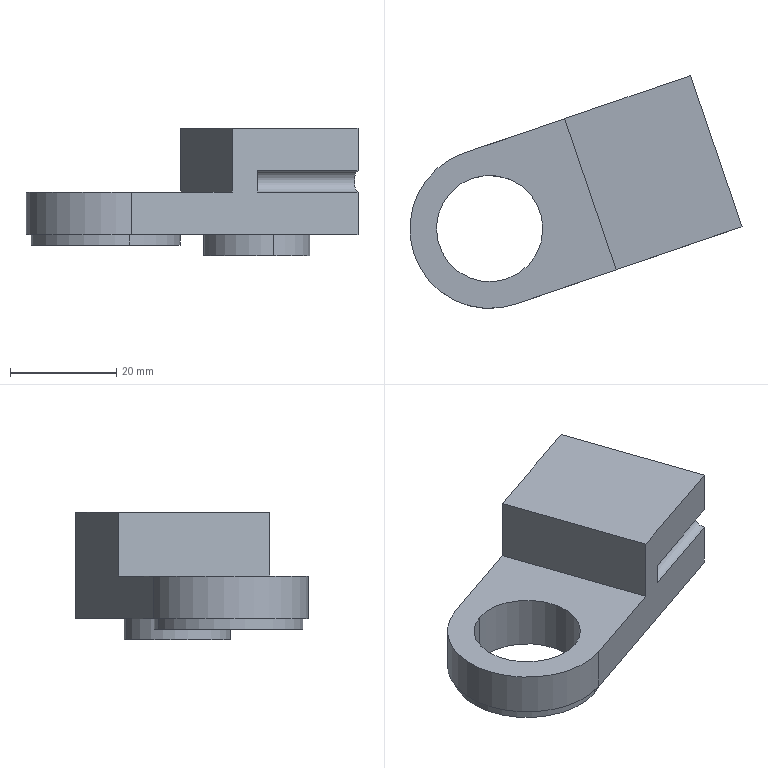Component | SolidWorks | SwingAssistFrame(Right)-2 | 1 solid | 21 faces | box 62.43 x 43.74 x 24 mm | volume 20749 mm3 | plane 11 | cylinder 10 | commonest cylinder face diameters 20 x4 10 x2 28 x2 30 x1 4 x1
build123d program:
from build123d import *
from build123d.topology import SkipClean

# Parameters (mm, degrees)
SKETCH1_2_R         = 10
BOSS_EXTRUDE1_DEPTH = 8
SKETCH2_W           = 30
SKETCH2_H           = 25
BOSS_EXTRUDE2_DEPTH = 12
SKETCH5_R           = 2
CUT_EXTRUDE2_DEPTH  = 20
BOSS_EXTRUDE6_START = 2
SKETCH12_R          = 14
SKETCH12_R_2        = 10
BOSS_EXTRUDE6_DEPTH = 2
SKETCH13_R          = 5
CUT_EXTRUDE5_DEPTH  = 10
LINKLAYERPAD_START  = 4
SKETCH1_R           = 10
SKETCH1_R_2         = 5
LINKLAYERPAD_DEPTH  = 4


with BuildPart() as part:
    # Sketch1_2 → Boss-Extrude1 (new body)
    with BuildSketch(Plane.XY):
        with BuildLine():
            Line((-15, 0), (-15, 45))
            Line((-15, 45), (15, 45))
            Line((15, 45), (15, 0))
            ThreePointArc((15, 0), (0, -15), (-15, 0))
        make_face()
        Circle(SKETCH1_2_R, mode=Mode.SUBTRACT)
    extrude(amount=BOSS_EXTRUDE1_DEPTH)

    # Sketch2 → Boss-Extrude2 (add)
    with BuildSketch(Plane.XY.offset(8)):
        with Locations((0, 32.5)):
            Rectangle(SKETCH2_W, SKETCH2_H)
    extrude(amount=BOSS_EXTRUDE2_DEPTH)

    # Sketch5 → Cut-Extrude2 (cut)
    with BuildSketch(Plane(origin=(0, 45, 0), x_dir=(1, 0, 0), z_dir=(0, 1, 0))):
        with Locations((15, -10)):
            Circle(SKETCH5_R)
    extrude(amount=-CUT_EXTRUDE2_DEPTH, mode=Mode.SUBTRACT)

    # Sketch12 → Boss-Extrude6 (add)
    with SkipClean():  # the faces are left unmerged after this step: merging them gives an invalid solid
        with BuildSketch(Plane(origin=(0, 0, 0), x_dir=(-1, 0, 0), z_dir=(0, 0, -1)).offset(BOSS_EXTRUDE6_START)):
            Circle(SKETCH12_R)
            Circle(SKETCH12_R_2, mode=Mode.SUBTRACT)
        extrude(amount=-BOSS_EXTRUDE6_DEPTH)

    # Sketch13 → Cut-Extrude5 (cut)
    with SkipClean():  # the faces are left unmerged after this step: merging them gives an invalid solid
        with BuildSketch(Plane(origin=(0, 0, 0), x_dir=(-1, 0, 0), z_dir=(0, 0, -1))):
            with Locations((0, 30)):
                Circle(SKETCH13_R)
        extrude(amount=-CUT_EXTRUDE5_DEPTH, mode=Mode.SUBTRACT)

    # Sketch1 → LinkLayerPad (add)
    with SkipClean():  # the faces are left unmerged after this step: merging them gives an invalid solid
        with BuildSketch(Plane(origin=(0, 0, 0), x_dir=(-1, 0, 0), z_dir=(0, 0, -1)).offset(LINKLAYERPAD_START)):
            with Locations(Location((0, 30, 0), (0, 0, 180))):
                Circle(SKETCH1_R)
            with Locations((0, 30)):
                Circle(SKETCH1_R_2, mode=Mode.SUBTRACT)
        extrude(amount=-LINKLAYERPAD_DEPTH)


solid = part.part

# Placed as in the assembly
solid = solid.moved(Location((17.47, 39.391, 116.846), (0, 0, -71.149)))
STEP:
#1=COLOUR_RGB('',0.7922,0.8196,0.9333);
#2=FILL_AREA_STYLE_COLOUR('',#1);
#3=FILL_AREA_STYLE('',(#2));
#4=SURFACE_STYLE_FILL_AREA(#3);
#5=SURFACE_SIDE_STYLE('',(#4));
#6=SURFACE_STYLE_USAGE(.BOTH.,#5);
#7=PRESENTATION_STYLE_ASSIGNMENT((#6));
#8=CARTESIAN_POINT('',(1.869,1.746,4.994));
#9=VERTEX_POINT('',#8);
#10=CARTESIAN_POINT('',(1.742,2.119,4.994));
#11=VERTEX_POINT('',#10);
#12=CARTESIAN_POINT('',(1.806,1.932,4.994));
#13=DIRECTION('',(-0.,0.,-1.));
#14=DIRECTION('',(-0.3231,0.9464,0.));
#15=AXIS2_PLACEMENT_3D('',#12,#13,#14);
#16=CIRCLE('',#15,0.1969);
#17=EDGE_CURVE('',#9,#11,#16,.T.);
#18=ORIENTED_EDGE('',*,*,#17,.F.);
#19=CARTESIAN_POINT('',(1.869,1.746,4.443));
#20=VERTEX_POINT('',#19);
#21=CARTESIAN_POINT('',(1.869,1.746,4.994));
#22=DIRECTION('',(-0.,0.,-1.));
#23=VECTOR('',#22,39.37);
#24=LINE('',#21,#23);
#25=EDGE_CURVE('',#9,#20,#24,.T.);
#26=ORIENTED_EDGE('',*,*,#25,.T.);
#27=CARTESIAN_POINT('',(1.742,2.119,4.443));
#28=VERTEX_POINT('',#27);
#29=CARTESIAN_POINT('',(1.806,1.932,4.443));
#30=DIRECTION('',(-0.,0.,-1.));
#31=DIRECTION('',(-0.3231,0.9464,0.));
#32=AXIS2_PLACEMENT_3D('',#29,#30,#31);
#33=CIRCLE('',#32,0.1969);
#34=EDGE_CURVE('',#20,#28,#33,.T.);
#35=ORIENTED_EDGE('',*,*,#34,.T.);
#36=CARTESIAN_POINT('',(1.742,2.119,4.994));
#37=DIRECTION('',(-0.,0.,-1.));
#38=VECTOR('',#37,39.37);
#39=LINE('',#36,#38);
#40=EDGE_CURVE('',#11,#28,#39,.T.);
#41=ORIENTED_EDGE('',*,*,#40,.F.);
#42=EDGE_LOOP('',(#18,#26,#35,#41));
#43=FACE_OUTER_BOUND('',#42,.T.);
#44=CARTESIAN_POINT('',(1.806,1.932,4.994));
#45=DIRECTION('',(-0.,0.,-1.));
#46=DIRECTION('',(-0.3231,0.9464,0.));
#47=AXIS2_PLACEMENT_3D('',#44,#45,#46);
#48=CYLINDRICAL_SURFACE('',#47,0.1969);
#49=ADVANCED_FACE('',(#43),#48,.F.);
#50=CARTESIAN_POINT('',(1.678,2.305,4.443));
#51=VERTEX_POINT('',#50);
#52=CARTESIAN_POINT('',(1.933,1.56,4.443));
#53=VERTEX_POINT('',#52);
#54=CARTESIAN_POINT('',(1.806,1.932,4.443));
#55=DIRECTION('',(-0.,0.,-1.));
#56=DIRECTION('',(-0.3231,0.9464,0.));
#57=AXIS2_PLACEMENT_3D('',#54,#55,#56);
#58=CIRCLE('',#57,0.3937);
#59=EDGE_CURVE('',#51,#53,#58,.T.);
#60=ORIENTED_EDGE('',*,*,#59,.F.);
#61=CARTESIAN_POINT('',(1.678,2.305,4.6));
#62=VERTEX_POINT('',#61);
#63=CARTESIAN_POINT('',(1.678,2.305,4.443));
#64=DIRECTION('',(0.,-0.,1.));
#65=VECTOR('',#64,39.37);
#66=LINE('',#63,#65);
#67=EDGE_CURVE('',#51,#62,#66,.T.);
#68=ORIENTED_EDGE('',*,*,#67,.T.);
#69=CARTESIAN_POINT('',(1.933,1.56,4.6));
#70=VERTEX_POINT('',#69);
#71=CARTESIAN_POINT('',(1.806,1.932,4.6));
#72=DIRECTION('',(-0.,0.,-1.));
#73=DIRECTION('',(0.3231,-0.9464,0.));
#74=AXIS2_PLACEMENT_3D('',#71,#72,#73);
#75=CIRCLE('',#74,0.3937);
#76=EDGE_CURVE('',#62,#70,#75,.T.);
#77=ORIENTED_EDGE('',*,*,#76,.T.);
#78=CARTESIAN_POINT('',(1.933,1.56,4.443));
#79=DIRECTION('',(0.,-0.,1.));
#80=VECTOR('',#79,39.37);
#81=LINE('',#78,#80);
#82=EDGE_CURVE('',#53,#70,#81,.T.);
#83=ORIENTED_EDGE('',*,*,#82,.F.);
#84=EDGE_LOOP('',(#60,#68,#77,#83));
#85=FACE_OUTER_BOUND('',#84,.T.);
#86=CARTESIAN_POINT('',(1.806,1.932,4.443));
#87=DIRECTION('',(0.,-0.,1.));
#88=DIRECTION('',(0.3231,-0.9464,0.));
#89=AXIS2_PLACEMENT_3D('',#86,#87,#88);
#90=CYLINDRICAL_SURFACE('',#89,0.3937);
#91=ADVANCED_FACE('',(#85),#90,.T.);
#92=CARTESIAN_POINT('',(0.5097,2.072,4.521));
#93=VERTEX_POINT('',#92);
#94=CARTESIAN_POINT('',(0.8659,1.029,4.521));
#95=VERTEX_POINT('',#94);
#96=CARTESIAN_POINT('',(0.6878,1.551,4.521));
#97=DIRECTION('',(-0.,0.,-1.));
#98=DIRECTION('',(-0.3231,0.9464,0.));
#99=AXIS2_PLACEMENT_3D('',#96,#97,#98);
#100=CIRCLE('',#99,0.5512);
#101=EDGE_CURVE('',#93,#95,#100,.T.);
#102=ORIENTED_EDGE('',*,*,#101,.F.);
#103=CARTESIAN_POINT('',(0.5097,2.072,4.6));
#104=VERTEX_POINT('',#103);
#105=CARTESIAN_POINT('',(0.5097,2.072,4.521));
#106=DIRECTION('',(0.,-0.,1.));
#107=VECTOR('',#106,39.37);
#108=LINE('',#105,#107);
#109=EDGE_CURVE('',#93,#104,#108,.T.);
#110=ORIENTED_EDGE('',*,*,#109,.T.);
#111=CARTESIAN_POINT('',(0.8659,1.029,4.6));
#112=VERTEX_POINT('',#111);
#113=CARTESIAN_POINT('',(0.6878,1.551,4.6));
#114=DIRECTION('',(-0.,0.,-1.));
#115=DIRECTION('',(-0.3231,0.9464,0.));
#116=AXIS2_PLACEMENT_3D('',#113,#114,#115);
#117=CIRCLE('',#116,0.5512);
#118=EDGE_CURVE('',#104,#112,#117,.T.);
#119=ORIENTED_EDGE('',*,*,#118,.T.);
#120=CARTESIAN_POINT('',(0.8659,1.029,4.521));
#121=DIRECTION('',(0.,-0.,1.));
#122=VECTOR('',#121,39.37);
#123=LINE('',#120,#122);
#124=EDGE_CURVE('',#95,#112,#123,.T.);
#125=ORIENTED_EDGE('',*,*,#124,.F.);
#126=EDGE_LOOP('',(#102,#110,#119,#125));
#127=FACE_OUTER_BOUND('',#126,.T.);
#128=CARTESIAN_POINT('',(0.6878,1.551,4.521));
#129=DIRECTION('',(0.,-0.,1.));
#130=DIRECTION('',(0.3231,-0.9464,0.));
#131=AXIS2_PLACEMENT_3D('',#128,#129,#130);
#132=CYLINDRICAL_SURFACE('',#131,0.5512);
#133=ADVANCED_FACE('',(#127),#132,.T.);
#134=CARTESIAN_POINT('',(0.5606,1.923,4.915));
#135=VERTEX_POINT('',#134);
#136=CARTESIAN_POINT('',(0.815,1.178,4.915));
#137=VERTEX_POINT('',#136);
#138=CARTESIAN_POINT('',(0.6878,1.551,4.915));
#139=DIRECTION('',(0.,-0.,1.));
#140=DIRECTION('',(0.3231,-0.9464,0.));
#141=AXIS2_PLACEMENT_3D('',#138,#139,#140);
#142=CIRCLE('',#141,0.3937);
#143=EDGE_CURVE('',#135,#137,#142,.T.);
#144=ORIENTED_EDGE('',*,*,#143,.T.);
#145=CARTESIAN_POINT('',(0.815,1.178,4.521));
#146=VERTEX_POINT('',#145);
#147=CARTESIAN_POINT('',(0.815,1.178,4.915));
#148=DIRECTION('',(-0.,0.,-1.));
#149=VECTOR('',#148,39.37);
#150=LINE('',#147,#149);
#151=EDGE_CURVE('',#137,#146,#150,.T.);
#152=ORIENTED_EDGE('',*,*,#151,.T.);
#153=CARTESIAN_POINT('',(0.5606,1.923,4.521));
#154=VERTEX_POINT('',#153);
#155=CARTESIAN_POINT('',(0.6878,1.551,4.521));
#156=DIRECTION('',(-0.,0.,-1.));
#157=DIRECTION('',(-0.3231,0.9464,0.));
#158=AXIS2_PLACEMENT_3D('',#155,#156,#157);
#159=CIRCLE('',#158,0.3937);
#160=EDGE_CURVE('',#146,#154,#159,.T.);
#161=ORIENTED_EDGE('',*,*,#160,.T.);
#162=CARTESIAN_POINT('',(0.5606,1.923,4.915));
#163=DIRECTION('',(-0.,0.,-1.));
#164=VECTOR('',#163,39.37);
#165=LINE('',#162,#164);
#166=EDGE_CURVE('',#135,#154,#165,.T.);
#167=ORIENTED_EDGE('',*,*,#166,.F.);
#168=EDGE_LOOP('',(#144,#152,#161,#167));
#169=FACE_OUTER_BOUND('',#168,.T.);
#170=CARTESIAN_POINT('',(0.6878,1.551,4.915));
#171=DIRECTION('',(-0.,0.,-1.));
#172=DIRECTION('',(-0.3231,0.9464,0.));
#173=AXIS2_PLACEMENT_3D('',#170,#171,#172);
#174=CYLINDRICAL_SURFACE('',#173,0.3937);
#175=ADVANCED_FACE('',(#169),#174,.F.);
#176=CARTESIAN_POINT('',(0.497,2.11,4.6));
#177=VERTEX_POINT('',#176);
#178=CARTESIAN_POINT('',(0.8786,0.992,4.6));
#179=VERTEX_POINT('',#178);
#180=CARTESIAN_POINT('',(0.6878,1.551,4.6));
#181=DIRECTION('',(0.,-0.,1.));
#182=DIRECTION('',(0.3231,-0.9464,0.));
#183=AXIS2_PLACEMENT_3D('',#180,#181,#182);
#184=CIRCLE('',#183,0.5906);
#185=EDGE_CURVE('',#177,#179,#184,.T.);
#186=ORIENTED_EDGE('',*,*,#185,.F.);
#187=CARTESIAN_POINT('',(2.174,2.682,4.6));
#188=VERTEX_POINT('',#187);
#189=CARTESIAN_POINT('',(0.497,2.11,4.6));
#190=DIRECTION('',(-0.9464,-0.3231,0.));
#191=VECTOR('',#190,39.37);
#192=LINE('',#189,#191);
#193=EDGE_CURVE('',#188,#177,#192,.T.);
#194=ORIENTED_EDGE('',*,*,#193,.F.);
#195=CARTESIAN_POINT('',(2.555,1.564,4.6));
#196=VERTEX_POINT('',#195);
#197=CARTESIAN_POINT('',(2.174,2.682,4.6));
#198=DIRECTION('',(-0.3231,0.9464,0.));
#199=VECTOR('',#198,39.37);
#200=LINE('',#197,#199);
#201=EDGE_CURVE('',#196,#188,#200,.T.);
#202=ORIENTED_EDGE('',*,*,#201,.F.);
#203=CARTESIAN_POINT('',(0.8786,0.992,4.6));
#204=DIRECTION('',(0.9464,0.3231,-0.));
#205=VECTOR('',#204,39.37);
#206=LINE('',#203,#205);
#207=EDGE_CURVE('',#179,#196,#206,.T.);
#208=ORIENTED_EDGE('',*,*,#207,.F.);
#209=EDGE_LOOP('',(#186,#194,#202,#208));
#210=FACE_OUTER_BOUND('',#209,.T.);
#211=CARTESIAN_POINT('',(0.6878,1.551,4.6));
#212=DIRECTION('',(-0.,0.,-1.));
#213=DIRECTION('',(-0.3231,0.9464,0.));
#214=AXIS2_PLACEMENT_3D('',#211,#212,#213);
#215=CIRCLE('',#214,0.5512);
#216=EDGE_CURVE('',#112,#104,#215,.T.);
#217=ORIENTED_EDGE('',*,*,#216,.F.);
#218=ORIENTED_EDGE('',*,*,#118,.F.);
#219=EDGE_LOOP('',(#217,#218));
#220=FACE_BOUND('',#219,.T.);
#221=CARTESIAN_POINT('',(1.806,1.932,4.6));
#222=DIRECTION('',(-0.,0.,-1.));
#223=DIRECTION('',(0.3231,-0.9464,0.));
#224=AXIS2_PLACEMENT_3D('',#221,#222,#223);
#225=CIRCLE('',#224,0.3937);
#226=EDGE_CURVE('',#70,#62,#225,.T.);
#227=ORIENTED_EDGE('',*,*,#226,.F.);
#228=ORIENTED_EDGE('',*,*,#76,.F.);
#229=EDGE_LOOP('',(#227,#228));
#230=FACE_BOUND('',#229,.T.);
#231=CARTESIAN_POINT('',(0.6878,1.551,4.6));
#232=DIRECTION('',(0.,-0.,1.));
#233=DIRECTION('',(0.3231,-0.9464,-0.));
#234=AXIS2_PLACEMENT_3D('',#231,#232,#233);
#235=PLANE('',#234);
#236=ADVANCED_FACE('',(#210,#220,#230),#235,.F.);
#237=CARTESIAN_POINT('',(1.242,2.364,4.915));
#238=VERTEX_POINT('',#237);
#239=CARTESIAN_POINT('',(1.624,1.246,4.915));
#240=VERTEX_POINT('',#239);
#241=CARTESIAN_POINT('',(1.242,2.364,4.915));
#242=DIRECTION('',(0.3231,-0.9464,-0.));
#243=VECTOR('',#242,39.37);
#244=LINE('',#241,#243);
#245=EDGE_CURVE('',#238,#240,#244,.T.);
#246=ORIENTED_EDGE('',*,*,#245,.F.);
#247=CARTESIAN_POINT('',(0.497,2.11,4.915));
#248=VERTEX_POINT('',#247);
#249=CARTESIAN_POINT('',(0.497,2.11,4.915));
#250=DIRECTION('',(-0.9464,-0.3231,0.));
#251=VECTOR('',#250,39.37);
#252=LINE('',#249,#251);
#253=EDGE_CURVE('',#238,#248,#252,.T.);
#254=ORIENTED_EDGE('',*,*,#253,.T.);
#255=CARTESIAN_POINT('',(0.8786,0.992,4.915));
#256=VERTEX_POINT('',#255);
#257=CARTESIAN_POINT('',(0.6878,1.551,4.915));
#258=DIRECTION('',(0.,-0.,1.));
#259=DIRECTION('',(0.3231,-0.9464,0.));
#260=AXIS2_PLACEMENT_3D('',#257,#258,#259);
#261=CIRCLE('',#260,0.5906);
#262=EDGE_CURVE('',#248,#256,#261,.T.);
#263=ORIENTED_EDGE('',*,*,#262,.T.);
#264=CARTESIAN_POINT('',(0.8786,0.992,4.915));
#265=DIRECTION('',(0.9464,0.3231,-0.));
#266=VECTOR('',#265,39.37);
#267=LINE('',#264,#266);
#268=EDGE_CURVE('',#256,#240,#267,.T.);
#269=ORIENTED_EDGE('',*,*,#268,.T.);
#270=EDGE_LOOP('',(#246,#254,#263,#269));
#271=FACE_OUTER_BOUND('',#270,.T.);
#272=ORIENTED_EDGE('',*,*,#143,.F.);
#273=CARTESIAN_POINT('',(0.6878,1.551,4.915));
#274=DIRECTION('',(0.,-0.,1.));
#275=DIRECTION('',(0.3231,-0.9464,0.));
#276=AXIS2_PLACEMENT_3D('',#273,#274,#275);
#277=CIRCLE('',#276,0.3937);
#278=EDGE_CURVE('',#137,#135,#277,.T.);
#279=ORIENTED_EDGE('',*,*,#278,.F.);
#280=EDGE_LOOP('',(#272,#279));
#281=FACE_BOUND('',#280,.T.);
#282=CARTESIAN_POINT('',(0.6878,1.551,4.915));
#283=DIRECTION('',(0.,-0.,1.));
#284=DIRECTION('',(0.3231,-0.9464,-0.));
#285=AXIS2_PLACEMENT_3D('',#282,#283,#284);
#286=PLANE('',#285);
#287=ADVANCED_FACE('',(#271,#281),#286,.T.);
#288=ORIENTED_EDGE('',*,*,#185,.T.);
#289=CARTESIAN_POINT('',(0.8786,0.992,4.915));
#290=DIRECTION('',(-0.,0.,-1.));
#291=VECTOR('',#290,39.37);
#292=LINE('',#289,#291);
#293=EDGE_CURVE('',#256,#179,#292,.T.);
#294=ORIENTED_EDGE('',*,*,#293,.F.);
#295=ORIENTED_EDGE('',*,*,#262,.F.);
#296=CARTESIAN_POINT('',(0.497,2.11,4.915));
#297=DIRECTION('',(-0.,0.,-1.));
#298=VECTOR('',#297,39.37);
#299=LINE('',#296,#298);
#300=EDGE_CURVE('',#248,#177,#299,.T.);
#301=ORIENTED_EDGE('',*,*,#300,.T.);
#302=EDGE_LOOP('',(#288,#294,#295,#301));
#303=FACE_OUTER_BOUND('',#302,.T.);
#304=CARTESIAN_POINT('',(0.6878,1.551,4.915));
#305=DIRECTION('',(-0.,0.,-1.));
#306=DIRECTION('',(-0.3231,0.9464,0.));
#307=AXIS2_PLACEMENT_3D('',#304,#305,#306);
#308=CYLINDRICAL_SURFACE('',#307,0.5906);
#309=ADVANCED_FACE('',(#303),#308,.T.);
#310=CARTESIAN_POINT('',(1.81,1.31,5.073));
#311=VERTEX_POINT('',#310);
#312=CARTESIAN_POINT('',(1.81,1.31,4.915));
#313=VERTEX_POINT('',#312);
#314=CARTESIAN_POINT('',(1.81,1.31,4.915));
#315=DIRECTION('',(-0.,0.,-1.));
#316=VECTOR('',#315,39.37);
#317=LINE('',#314,#316);
#318=EDGE_CURVE('',#311,#313,#317,.T.);
#319=ORIENTED_EDGE('',*,*,#318,.F.);
#320=CARTESIAN_POINT('',(2.555,1.564,5.073));
#321=VERTEX_POINT('',#320);
#322=CARTESIAN_POINT('',(1.81,1.31,5.073));
#323=DIRECTION('',(0.9464,0.3231,-0.));
#324=VECTOR('',#323,39.37);
#325=LINE('',#322,#324);
#326=EDGE_CURVE('',#311,#321,#325,.T.);
#327=ORIENTED_EDGE('',*,*,#326,.T.);
#328=CARTESIAN_POINT('',(2.555,1.564,5.388));
#329=VERTEX_POINT('',#328);
#330=CARTESIAN_POINT('',(2.555,1.564,4.915));
#331=DIRECTION('',(-0.,0.,-1.));
#332=VECTOR('',#331,39.37);
#333=LINE('',#330,#332);
#334=EDGE_CURVE('',#329,#321,#333,.T.);
#335=ORIENTED_EDGE('',*,*,#334,.F.);
#336=CARTESIAN_POINT('',(1.624,1.246,5.388));
#337=VERTEX_POINT('',#336);
#338=CARTESIAN_POINT('',(1.624,1.246,5.388));
#339=DIRECTION('',(0.9464,0.3231,-0.));
#340=VECTOR('',#339,39.37);
#341=LINE('',#338,#340);
#342=EDGE_CURVE('',#337,#329,#341,.T.);
#343=ORIENTED_EDGE('',*,*,#342,.F.);
#344=CARTESIAN_POINT('',(1.624,1.246,5.388));
#345=DIRECTION('',(-0.,0.,-1.));
#346=VECTOR('',#345,39.37);
#347=LINE('',#344,#346);
#348=EDGE_CURVE('',#337,#240,#347,.T.);
#349=ORIENTED_EDGE('',*,*,#348,.T.);
#350=ORIENTED_EDGE('',*,*,#268,.F.);
#351=ORIENTED_EDGE('',*,*,#293,.T.);
#352=ORIENTED_EDGE('',*,*,#207,.T.);
#353=CARTESIAN_POINT('',(2.555,1.564,4.915));
#354=VERTEX_POINT('',#353);
#355=CARTESIAN_POINT('',(2.555,1.564,4.915));
#356=DIRECTION('',(-0.,0.,-1.));
#357=VECTOR('',#356,39.37);
#358=LINE('',#355,#357);
#359=EDGE_CURVE('',#354,#196,#358,.T.);
#360=ORIENTED_EDGE('',*,*,#359,.F.);
#361=CARTESIAN_POINT('',(1.81,1.31,4.915));
#362=DIRECTION('',(-0.9464,-0.3231,0.));
#363=VECTOR('',#362,39.37);
#364=LINE('',#361,#363);
#365=EDGE_CURVE('',#354,#313,#364,.T.);
#366=ORIENTED_EDGE('',*,*,#365,.T.);
#367=EDGE_LOOP('',(#319,#327,#335,#343,#349,#350,#351,#352,#360,#366));
#368=FACE_OUTER_BOUND('',#367,.T.);
#369=CARTESIAN_POINT('',(0.8786,0.992,4.915));
#370=DIRECTION('',(-0.3231,0.9464,0.));
#371=DIRECTION('',(0.,-0.,1.));
#372=AXIS2_PLACEMENT_3D('',#369,#370,#371);
#373=PLANE('',#372);
#374=ADVANCED_FACE('',(#368),#373,.F.);
#375=ORIENTED_EDGE('',*,*,#334,.T.);
#376=CARTESIAN_POINT('',(2.555,1.564,4.994));
#377=DIRECTION('',(-0.9464,-0.3231,0.));
#378=DIRECTION('',(0.,0.,-1.));
#379=AXIS2_PLACEMENT_3D('',#376,#377,#378);
#380=CIRCLE('',#379,0.07874);
#381=EDGE_CURVE('',#321,#354,#380,.T.);
#382=ORIENTED_EDGE('',*,*,#381,.T.);
#383=ORIENTED_EDGE('',*,*,#359,.T.);
#384=ORIENTED_EDGE('',*,*,#201,.T.);
#385=CARTESIAN_POINT('',(2.174,2.682,5.388));
#386=VERTEX_POINT('',#385);
#387=CARTESIAN_POINT('',(2.174,2.682,4.915));
#388=DIRECTION('',(-0.,0.,-1.));
#389=VECTOR('',#388,39.37);
#390=LINE('',#387,#389);
#391=EDGE_CURVE('',#386,#188,#390,.T.);
#392=ORIENTED_EDGE('',*,*,#391,.F.);
#393=CARTESIAN_POINT('',(2.555,1.564,5.388));
#394=DIRECTION('',(-0.3231,0.9464,0.));
#395=VECTOR('',#394,39.37);
#396=LINE('',#393,#395);
#397=EDGE_CURVE('',#329,#386,#396,.T.);
#398=ORIENTED_EDGE('',*,*,#397,.F.);
#399=EDGE_LOOP('',(#375,#382,#383,#384,#392,#398));
#400=FACE_OUTER_BOUND('',#399,.T.);
#401=CARTESIAN_POINT('',(2.174,2.682,4.915));
#402=DIRECTION('',(-0.9464,-0.3231,0.));
#403=DIRECTION('',(-0.,0.,-1.));
#404=AXIS2_PLACEMENT_3D('',#401,#402,#403);
#405=PLANE('',#404);
#406=ADVANCED_FACE('',(#400),#405,.F.);
#407=ORIENTED_EDGE('',*,*,#193,.T.);
#408=ORIENTED_EDGE('',*,*,#300,.F.);
#409=ORIENTED_EDGE('',*,*,#253,.F.);
#410=CARTESIAN_POINT('',(1.242,2.364,5.388));
#411=VERTEX_POINT('',#410);
#412=CARTESIAN_POINT('',(1.242,2.364,5.388));
#413=DIRECTION('',(-0.,0.,-1.));
#414=VECTOR('',#413,39.37);
#415=LINE('',#412,#414);
#416=EDGE_CURVE('',#411,#238,#415,.T.);
#417=ORIENTED_EDGE('',*,*,#416,.F.);
#418=CARTESIAN_POINT('',(2.174,2.682,5.388));
#419=DIRECTION('',(-0.9464,-0.3231,0.));
#420=VECTOR('',#419,39.37);
#421=LINE('',#418,#420);
#422=EDGE_CURVE('',#386,#411,#421,.T.);
#423=ORIENTED_EDGE('',*,*,#422,.F.);
#424=ORIENTED_EDGE('',*,*,#391,.T.);
#425=EDGE_LOOP('',(#407,#408,#409,#417,#423,#424));
#426=FACE_OUTER_BOUND('',#425,.T.);
#427=CARTESIAN_POINT('',(0.497,2.11,4.915));
#428=DIRECTION('',(0.3231,-0.9464,-0.));
#429=DIRECTION('',(-0.,0.,-1.));
#430=AXIS2_PLACEMENT_3D('',#427,#428,#429);
#431=PLANE('',#430);
#432=ADVANCED_FACE('',(#426),#431,.F.);
#433=ORIENTED_EDGE('',*,*,#151,.F.);
#434=ORIENTED_EDGE('',*,*,#278,.T.);
#435=ORIENTED_EDGE('',*,*,#166,.T.);
#436=CARTESIAN_POINT('',(0.6878,1.551,4.521));
#437=DIRECTION('',(-0.,0.,-1.));
#438=DIRECTION('',(-0.3231,0.9464,0.));
#439=AXIS2_PLACEMENT_3D('',#436,#437,#438);
#440=CIRCLE('',#439,0.3937);
#441=EDGE_CURVE('',#154,#146,#440,.T.);
#442=ORIENTED_EDGE('',*,*,#441,.T.);
#443=EDGE_LOOP('',(#433,#434,#435,#442));
#444=FACE_OUTER_BOUND('',#443,.T.);
#445=CARTESIAN_POINT('',(0.6878,1.551,4.915));
#446=DIRECTION('',(-0.,0.,-1.));
#447=DIRECTION('',(-0.3231,0.9464,0.));
#448=AXIS2_PLACEMENT_3D('',#445,#446,#447);
#449=CYLINDRICAL_SURFACE('',#448,0.3937);
#450=ADVANCED_FACE('',(#444),#449,.F.);
#451=ORIENTED_EDGE('',*,*,#245,.T.);
#452=ORIENTED_EDGE('',*,*,#348,.F.);
#453=CARTESIAN_POINT('',(1.242,2.364,5.388));
#454=DIRECTION('',(0.3231,-0.9464,-0.));
#455=VECTOR('',#454,39.37);
#456=LINE('',#453,#455);
#457=EDGE_CURVE('',#411,#337,#456,.T.);
#458=ORIENTED_EDGE('',*,*,#457,.F.);
#459=ORIENTED_EDGE('',*,*,#416,.T.);
#460=EDGE_LOOP('',(#451,#452,#458,#459));
#461=FACE_OUTER_BOUND('',#460,.T.);
#462=CARTESIAN_POINT('',(1.242,2.364,5.388));
#463=DIRECTION('',(0.9464,0.3231,-0.));
#464=DIRECTION('',(0.,-0.,1.));
#465=AXIS2_PLACEMENT_3D('',#462,#463,#464);
#466=PLANE('',#465);
#467=ADVANCED_FACE('',(#461),#466,.F.);
#468=ORIENTED_EDGE('',*,*,#397,.T.);
#469=ORIENTED_EDGE('',*,*,#422,.T.);
#470=ORIENTED_EDGE('',*,*,#457,.T.);
#471=ORIENTED_EDGE('',*,*,#342,.T.);
#472=EDGE_LOOP('',(#468,#469,#470,#471));
#473=FACE_OUTER_BOUND('',#472,.T.);
#474=CARTESIAN_POINT('',(0.6878,1.551,5.388));
#475=DIRECTION('',(0.,-0.,1.));
#476=DIRECTION('',(0.3231,-0.9464,-0.));
#477=AXIS2_PLACEMENT_3D('',#474,#475,#476);
#478=PLANE('',#477);
#479=ADVANCED_FACE('',(#473),#478,.T.);
#480=ORIENTED_EDGE('',*,*,#318,.T.);
#481=CARTESIAN_POINT('',(1.81,1.31,4.994));
#482=DIRECTION('',(0.9464,0.3231,-0.));
#483=DIRECTION('',(0.,0.,1.));
#484=AXIS2_PLACEMENT_3D('',#481,#482,#483);
#485=CIRCLE('',#484,0.07874);
#486=EDGE_CURVE('',#313,#311,#485,.T.);
#487=ORIENTED_EDGE('',*,*,#486,.T.);
#488=EDGE_LOOP('',(#480,#487));
#489=FACE_OUTER_BOUND('',#488,.T.);
#490=CARTESIAN_POINT('',(1.81,1.31,4.994));
#491=DIRECTION('',(0.9464,0.3231,-0.));
#492=DIRECTION('',(0.,-0.,1.));
#493=AXIS2_PLACEMENT_3D('',#490,#491,#492);
#494=PLANE('',#493);
#495=ADVANCED_FACE('',(#489),#494,.T.);
#496=ORIENTED_EDGE('',*,*,#486,.F.);
#497=ORIENTED_EDGE('',*,*,#365,.F.);
#498=ORIENTED_EDGE('',*,*,#381,.F.);
#499=ORIENTED_EDGE('',*,*,#326,.F.);
#500=EDGE_LOOP('',(#496,#497,#498,#499));
#501=FACE_OUTER_BOUND('',#500,.T.);
#502=CARTESIAN_POINT('',(1.81,1.31,4.994));
#503=DIRECTION('',(0.9464,0.3231,-0.));
#504=DIRECTION('',(0.,0.,1.));
#505=AXIS2_PLACEMENT_3D('',#502,#503,#504);
#506=CYLINDRICAL_SURFACE('',#505,0.07874);
#507=ADVANCED_FACE('',(#501),#506,.F.);
#508=CARTESIAN_POINT('',(0.6878,1.551,4.521));
#509=DIRECTION('',(-0.,0.,-1.));
#510=DIRECTION('',(-0.3231,0.9464,0.));
#511=AXIS2_PLACEMENT_3D('',#508,#509,#510);
#512=CIRCLE('',#511,0.5512);
#513=EDGE_CURVE('',#95,#93,#512,.T.);
#514=ORIENTED_EDGE('',*,*,#513,.T.);
#515=ORIENTED_EDGE('',*,*,#101,.T.);
#516=EDGE_LOOP('',(#514,#515));
#517=FACE_OUTER_BOUND('',#516,.T.);
#518=ORIENTED_EDGE('',*,*,#441,.F.);
#519=ORIENTED_EDGE('',*,*,#160,.F.);
#520=EDGE_LOOP('',(#518,#519));
#521=FACE_BOUND('',#520,.T.);
#522=CARTESIAN_POINT('',(0.6878,1.551,4.521));
#523=DIRECTION('',(-0.,0.,-1.));
#524=DIRECTION('',(-0.3231,0.9464,0.));
#525=AXIS2_PLACEMENT_3D('',#522,#523,#524);
#526=PLANE('',#525);
#527=ADVANCED_FACE('',(#517,#521),#526,.T.);
#528=ORIENTED_EDGE('',*,*,#109,.F.);
#529=ORIENTED_EDGE('',*,*,#513,.F.);
#530=ORIENTED_EDGE('',*,*,#124,.T.);
#531=ORIENTED_EDGE('',*,*,#216,.T.);
#532=EDGE_LOOP('',(#528,#529,#530,#531));
#533=FACE_OUTER_BOUND('',#532,.T.);
#534=CARTESIAN_POINT('',(0.6878,1.551,4.521));
#535=DIRECTION('',(0.,-0.,1.));
#536=DIRECTION('',(0.3231,-0.9464,0.));
#537=AXIS2_PLACEMENT_3D('',#534,#535,#536);
#538=CYLINDRICAL_SURFACE('',#537,0.5512);
#539=ADVANCED_FACE('',(#533),#538,.T.);
#540=CARTESIAN_POINT('',(1.806,1.932,4.443));
#541=DIRECTION('',(-0.,0.,-1.));
#542=DIRECTION('',(-0.3231,0.9464,0.));
#543=AXIS2_PLACEMENT_3D('',#540,#541,#542);
#544=CIRCLE('',#543,0.3937);
#545=EDGE_CURVE('',#53,#51,#544,.T.);
#546=ORIENTED_EDGE('',*,*,#545,.T.);
#547=ORIENTED_EDGE('',*,*,#59,.T.);
#548=EDGE_LOOP('',(#546,#547));
#549=FACE_OUTER_BOUND('',#548,.T.);
#550=CARTESIAN_POINT('',(1.806,1.932,4.443));
#551=DIRECTION('',(-0.,0.,-1.));
#552=DIRECTION('',(-0.3231,0.9464,0.));
#553=AXIS2_PLACEMENT_3D('',#550,#551,#552);
#554=CIRCLE('',#553,0.1969);
#555=EDGE_CURVE('',#28,#20,#554,.T.);
#556=ORIENTED_EDGE('',*,*,#555,.F.);
#557=ORIENTED_EDGE('',*,*,#34,.F.);
#558=EDGE_LOOP('',(#556,#557));
#559=FACE_BOUND('',#558,.T.);
#560=CARTESIAN_POINT('',(1.806,1.932,4.443));
#561=DIRECTION('',(-0.,0.,-1.));
#562=DIRECTION('',(-0.3231,0.9464,0.));
#563=AXIS2_PLACEMENT_3D('',#560,#561,#562);
#564=PLANE('',#563);
#565=ADVANCED_FACE('',(#549,#559),#564,.T.);
#566=ORIENTED_EDGE('',*,*,#67,.F.);
#567=ORIENTED_EDGE('',*,*,#545,.F.);
#568=ORIENTED_EDGE('',*,*,#82,.T.);
#569=ORIENTED_EDGE('',*,*,#226,.T.);
#570=EDGE_LOOP('',(#566,#567,#568,#569));
#571=FACE_OUTER_BOUND('',#570,.T.);
#572=CARTESIAN_POINT('',(1.806,1.932,4.443));
#573=DIRECTION('',(0.,-0.,1.));
#574=DIRECTION('',(0.3231,-0.9464,0.));
#575=AXIS2_PLACEMENT_3D('',#572,#573,#574);
#576=CYLINDRICAL_SURFACE('',#575,0.3937);
#577=ADVANCED_FACE('',(#571),#576,.T.);
#578=CARTESIAN_POINT('',(1.806,1.932,4.994));
#579=DIRECTION('',(-0.,0.,-1.));
#580=DIRECTION('',(-0.3231,0.9464,0.));
#581=AXIS2_PLACEMENT_3D('',#578,#579,#580);
#582=CIRCLE('',#581,0.1969);
#583=EDGE_CURVE('',#11,#9,#582,.T.);
#584=ORIENTED_EDGE('',*,*,#583,.T.);
#585=ORIENTED_EDGE('',*,*,#17,.T.);
#586=EDGE_LOOP('',(#584,#585));
#587=FACE_OUTER_BOUND('',#586,.T.);
#588=CARTESIAN_POINT('',(1.806,1.932,4.994));
#589=DIRECTION('',(-0.,0.,-1.));
#590=DIRECTION('',(-0.3231,0.9464,0.));
#591=AXIS2_PLACEMENT_3D('',#588,#589,#590);
#592=PLANE('',#591);
#593=ADVANCED_FACE('',(#587),#592,.T.);
#594=ORIENTED_EDGE('',*,*,#25,.F.);
#595=ORIENTED_EDGE('',*,*,#583,.F.);
#596=ORIENTED_EDGE('',*,*,#40,.T.);
#597=ORIENTED_EDGE('',*,*,#555,.T.);
#598=EDGE_LOOP('',(#594,#595,#596,#597));
#599=FACE_OUTER_BOUND('',#598,.T.);
#600=CARTESIAN_POINT('',(1.806,1.932,4.994));
#601=DIRECTION('',(-0.,0.,-1.));
#602=DIRECTION('',(-0.3231,0.9464,0.));
#603=AXIS2_PLACEMENT_3D('',#600,#601,#602);
#604=CYLINDRICAL_SURFACE('',#603,0.1969);
#605=ADVANCED_FACE('',(#599),#604,.F.);
#606=CLOSED_SHELL('',(#49,#91,#133,#175,#236,#287,#309,#374,#406,#432,#450,#467,#479,#495,#507,#527,#539,#565,#577,#593,#605));
#607=MANIFOLD_SOLID_BREP('',#606);
#608=STYLED_ITEM('',(#7),#607);
#609=(LENGTH_UNIT()NAMED_UNIT(*)SI_UNIT($,.METRE.));
#610=LENGTH_MEASURE_WITH_UNIT(LENGTH_MEASURE(0.0254),#609);
#611=DIMENSIONAL_EXPONENTS(1.,0.,0.,0.,0.,0.,0.);
#612=(CONVERSION_BASED_UNIT('',#610)LENGTH_UNIT()NAMED_UNIT(#611));
#613=UNCERTAINTY_MEASURE_WITH_UNIT(LENGTH_MEASURE(0.00001),#612,'','');
#614=(NAMED_UNIT(*)PLANE_ANGLE_UNIT()SI_UNIT($,.RADIAN.));
#615=(NAMED_UNIT(*)SI_UNIT($,.STERADIAN.)SOLID_ANGLE_UNIT());
#616=(GEOMETRIC_REPRESENTATION_CONTEXT(3)GLOBAL_UNCERTAINTY_ASSIGNED_CONTEXT((#613))GLOBAL_UNIT_ASSIGNED_CONTEXT((#612,#614,#615))REPRESENTATION_CONTEXT('',''));
#617=MECHANICAL_DESIGN_GEOMETRIC_PRESENTATION_REPRESENTATION('',(#608),#616);
#618=CARTESIAN_POINT('',(0.,0.,0.));
#619=DIRECTION('',(0.,0.,1.));
#620=DIRECTION('',(1.,0.,0.));
#621=AXIS2_PLACEMENT_3D('',#618,#619,#620);
#622=(LENGTH_UNIT()NAMED_UNIT(*)SI_UNIT($,.METRE.));
#623=LENGTH_MEASURE_WITH_UNIT(LENGTH_MEASURE(0.0254),#622);
#624=DIMENSIONAL_EXPONENTS(1.,0.,0.,0.,0.,0.,0.);
#625=(CONVERSION_BASED_UNIT('',#623)LENGTH_UNIT()NAMED_UNIT(#624));
#626=UNCERTAINTY_MEASURE_WITH_UNIT(LENGTH_MEASURE(0.00001),#625,'','');
#627=(NAMED_UNIT(*)PLANE_ANGLE_UNIT()SI_UNIT($,.RADIAN.));
#628=(NAMED_UNIT(*)SI_UNIT($,.STERADIAN.)SOLID_ANGLE_UNIT());
#629=(GEOMETRIC_REPRESENTATION_CONTEXT(3)GLOBAL_UNCERTAINTY_ASSIGNED_CONTEXT((#626))GLOBAL_UNIT_ASSIGNED_CONTEXT((#625,#627,#628))REPRESENTATION_CONTEXT('',''));
#630=ADVANCED_BREP_SHAPE_REPRESENTATION('',(#607,#621),#629);
#631=PRESENTATION_LAYER_ASSIGNMENT('','',(#608));